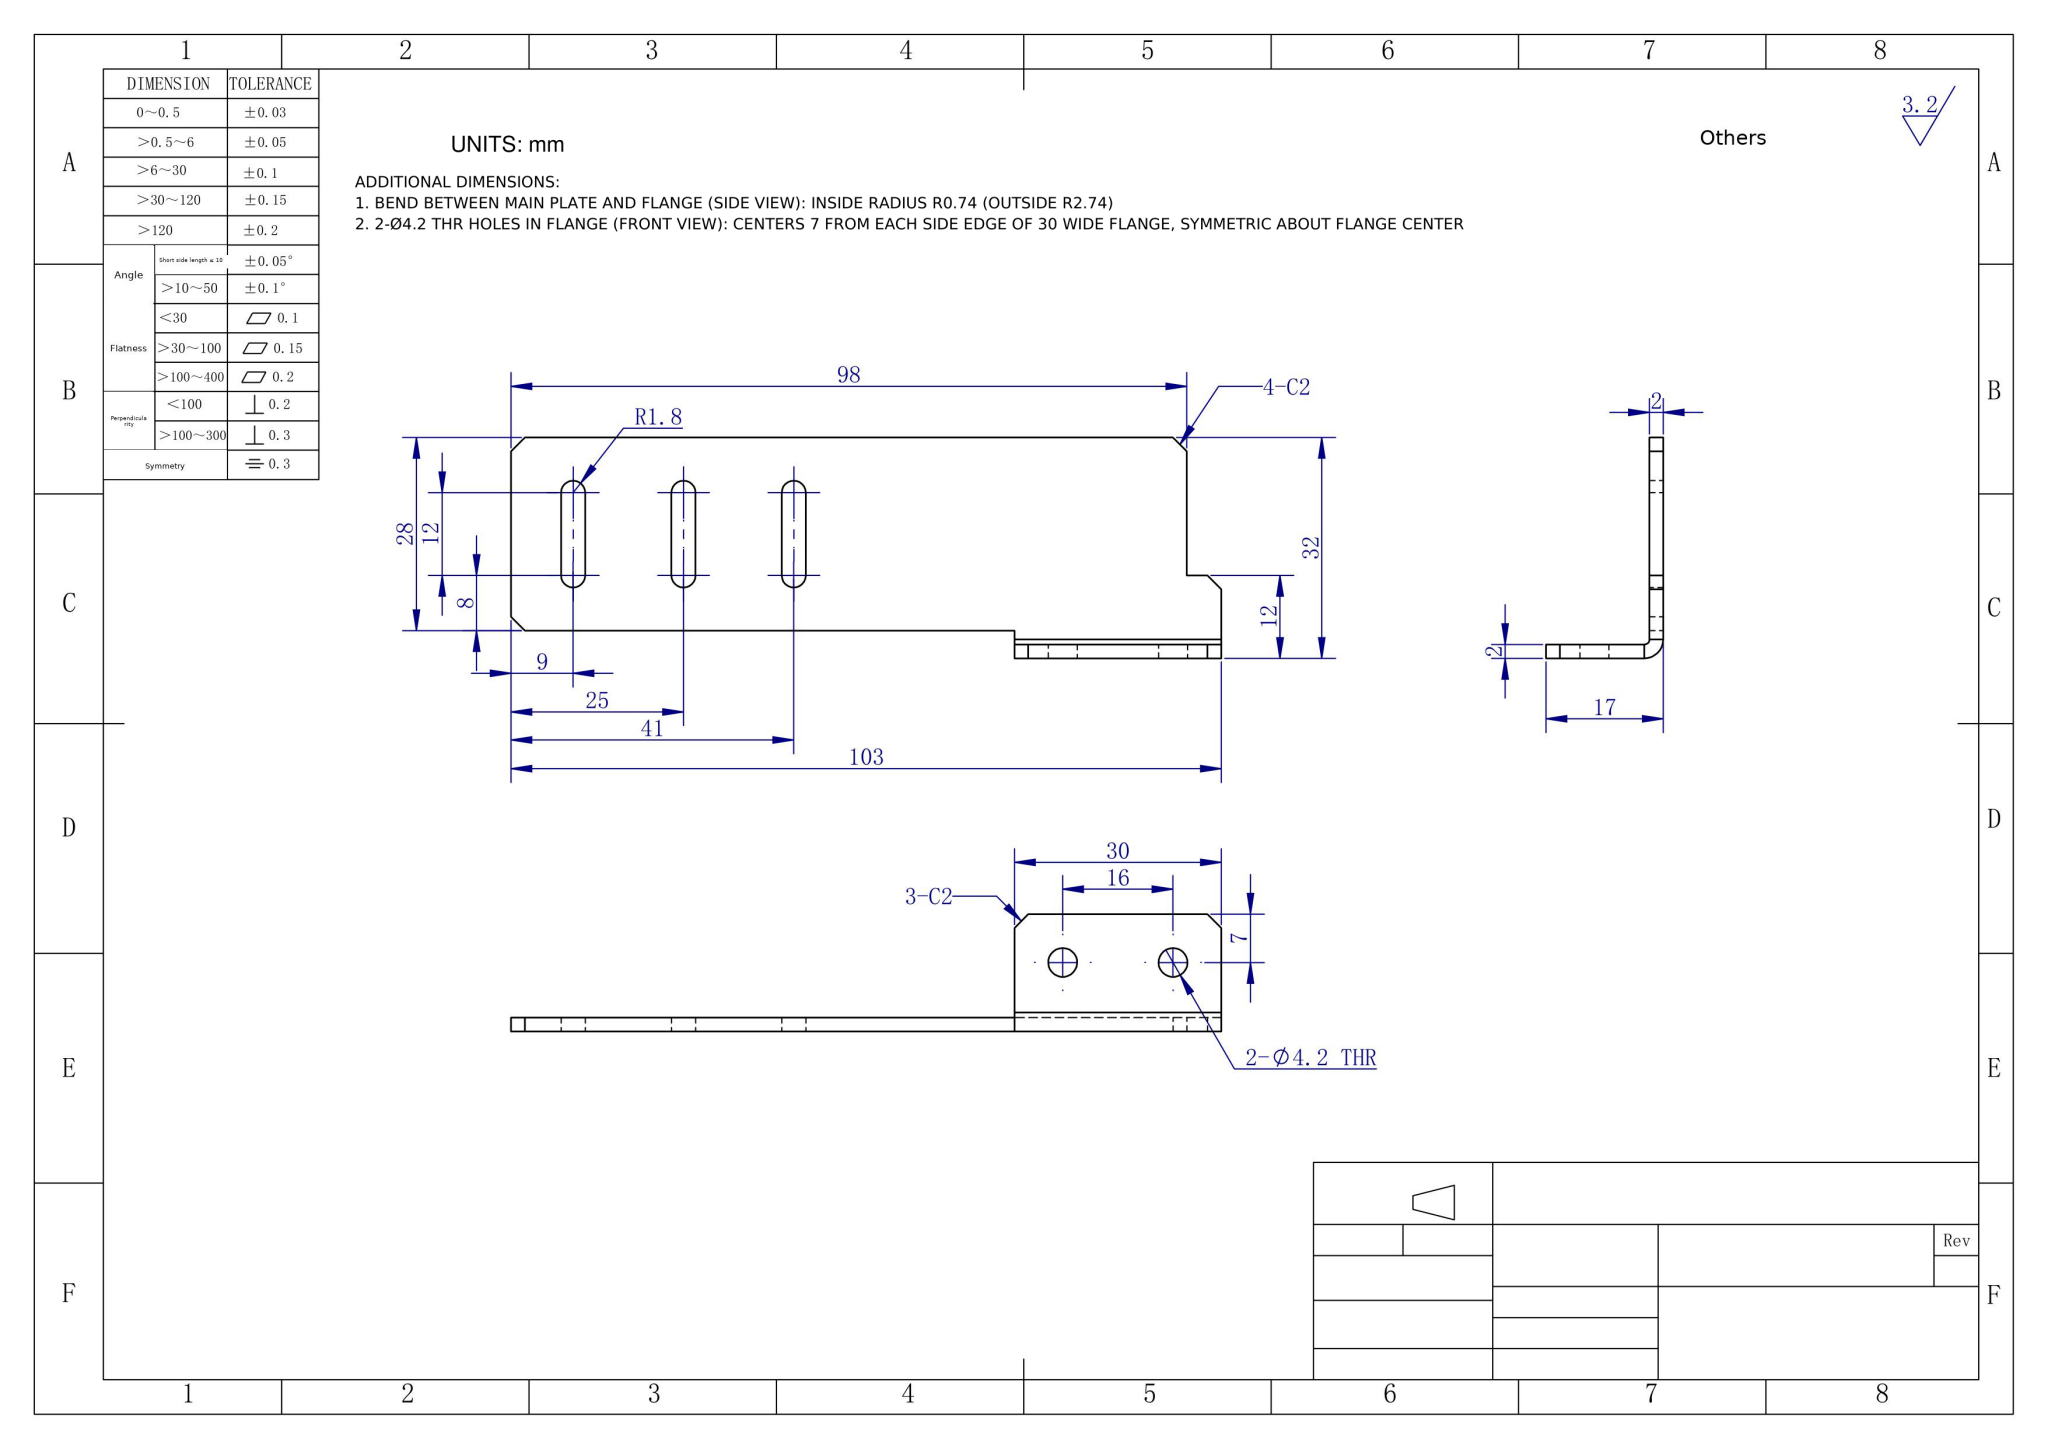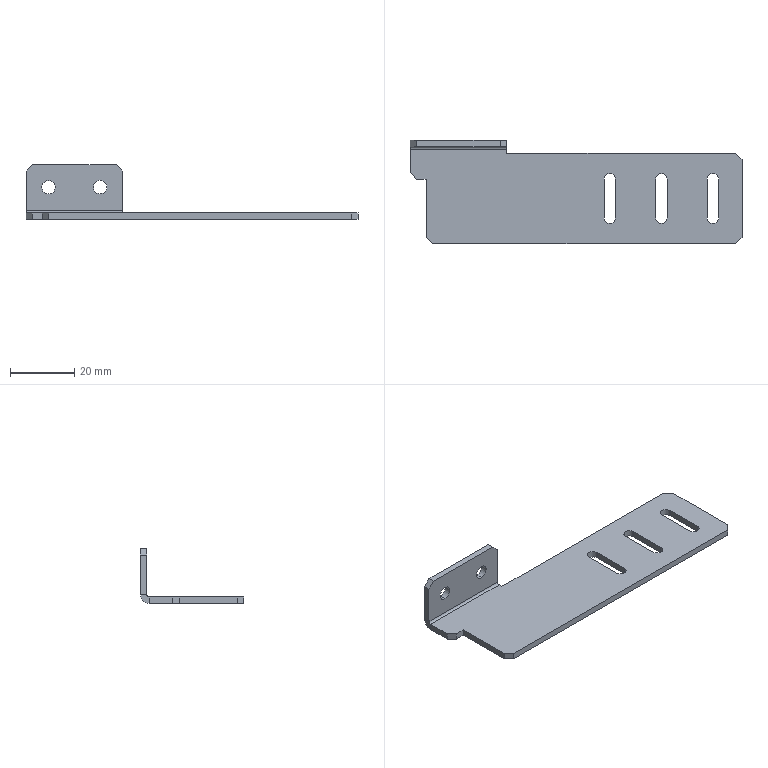Part | NX | mm | 1 solid | 40 faces | box 103 x 32 x 17 mm | volume 6274 mm3 | plane 28 | cylinder 12 | commonest cylinder face diameters 3.5 x6 4.2 x4 5.473 x1 1.473 x1